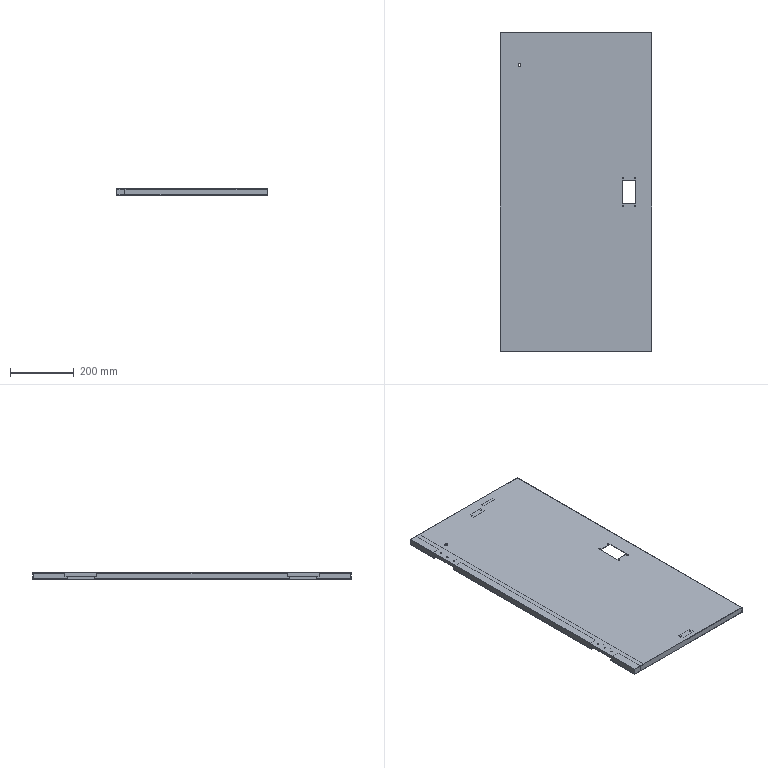Component | SolidWorks | SYM0671-81-200-1_SYM0671-81-201-1 | 1 solid | 108 faces | volume 953755 mm3 | plane 74 | cylinder 34 | commonest cylinder face diameters 3 x12 4 x12 5 x8 9 x2 | material Steel